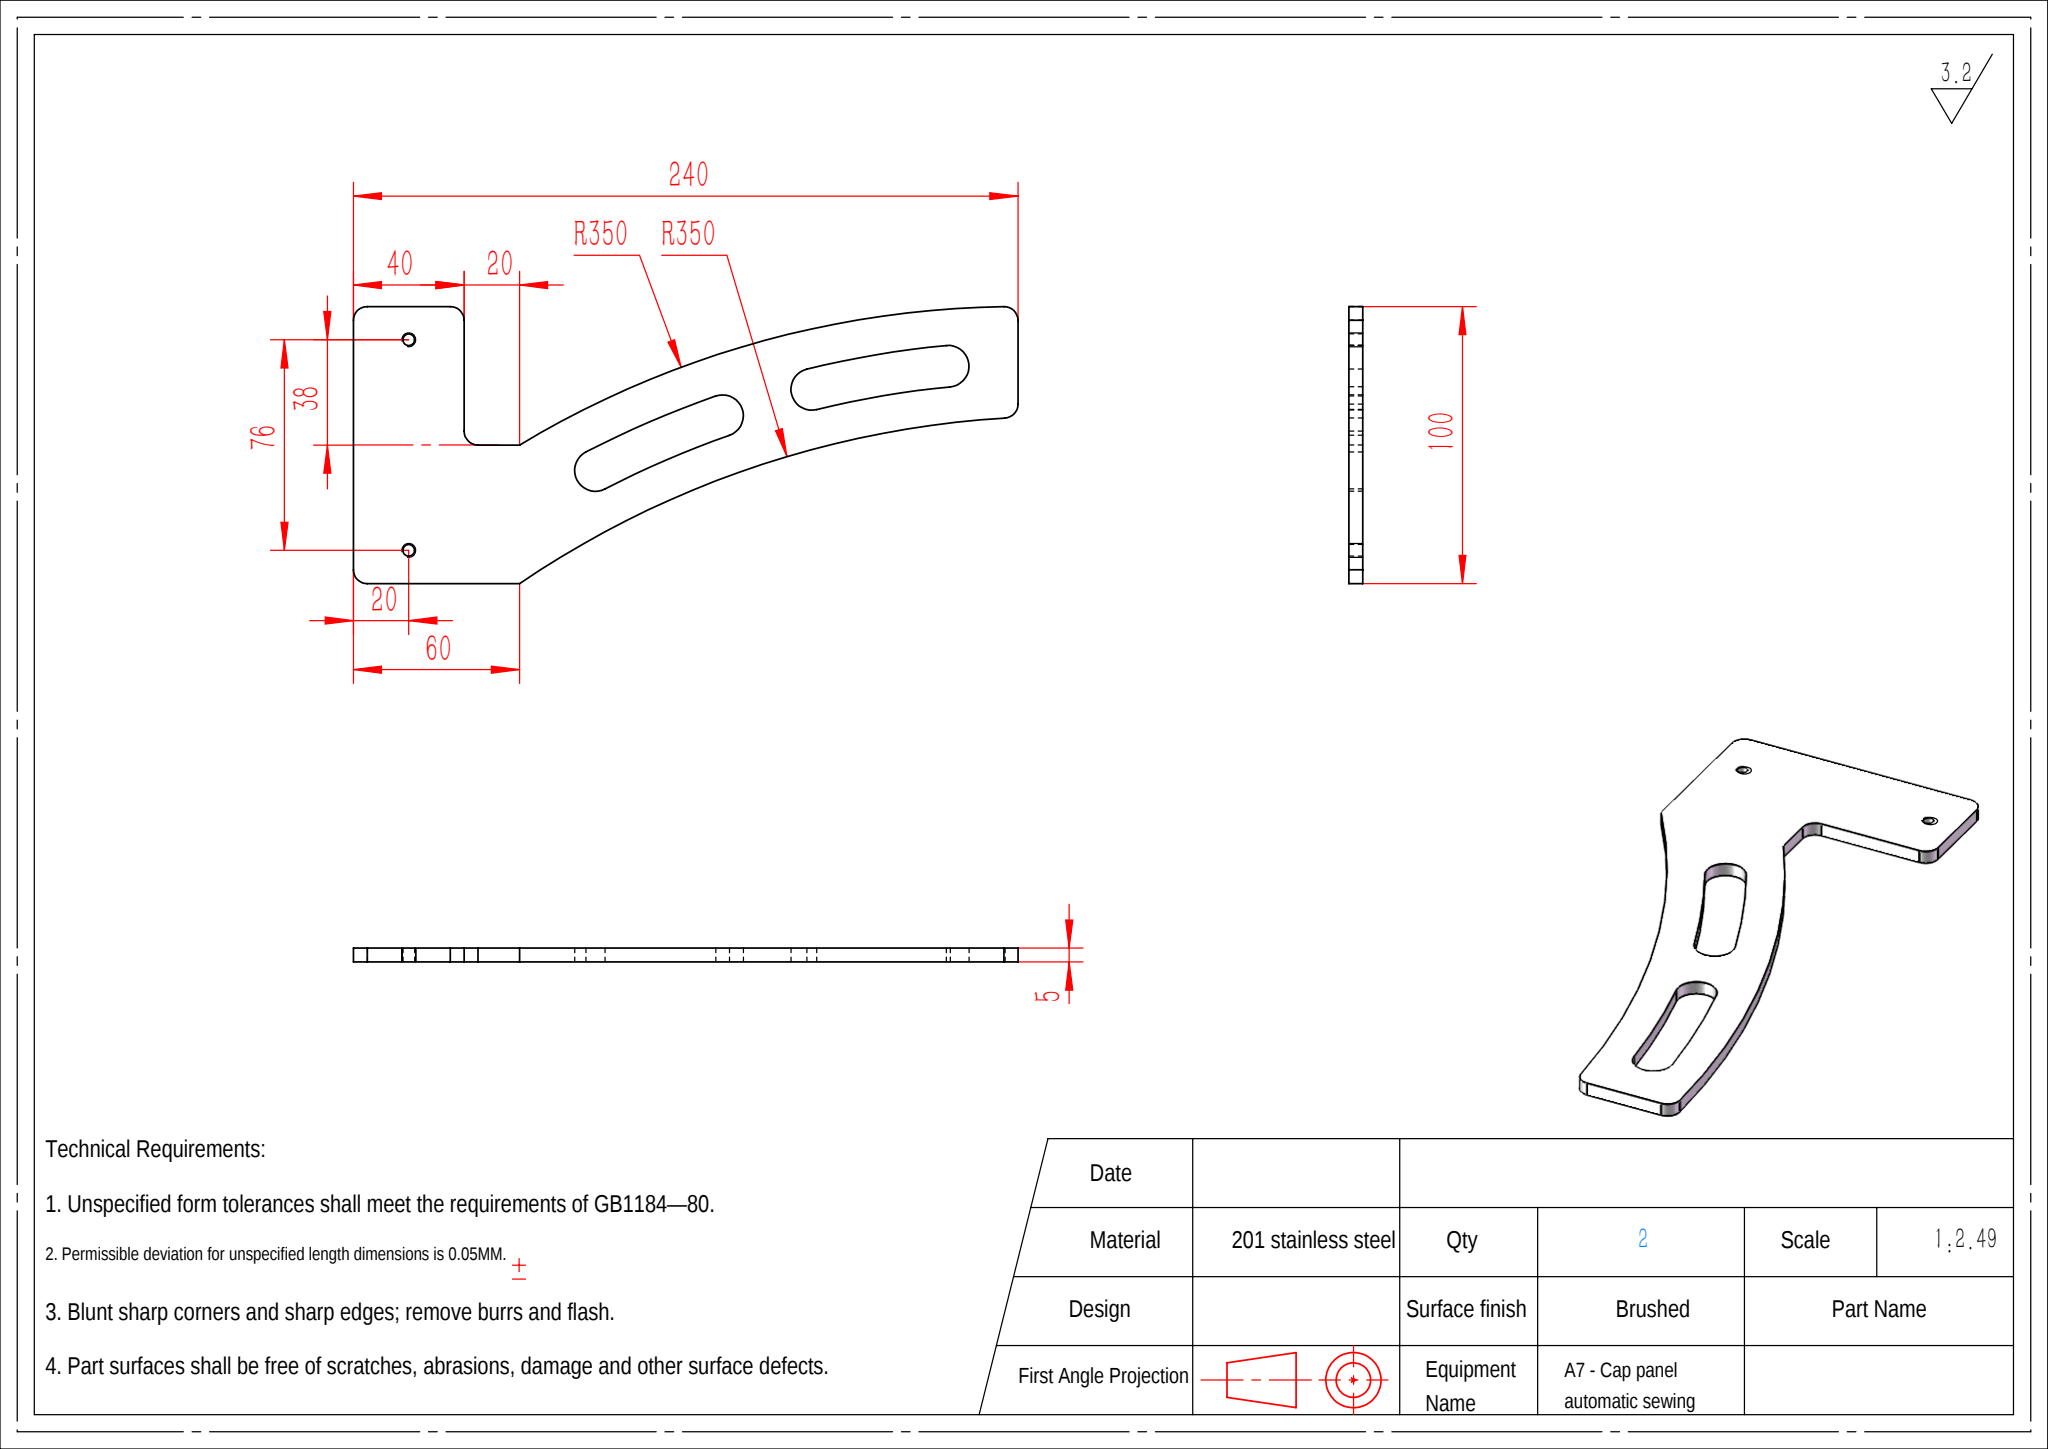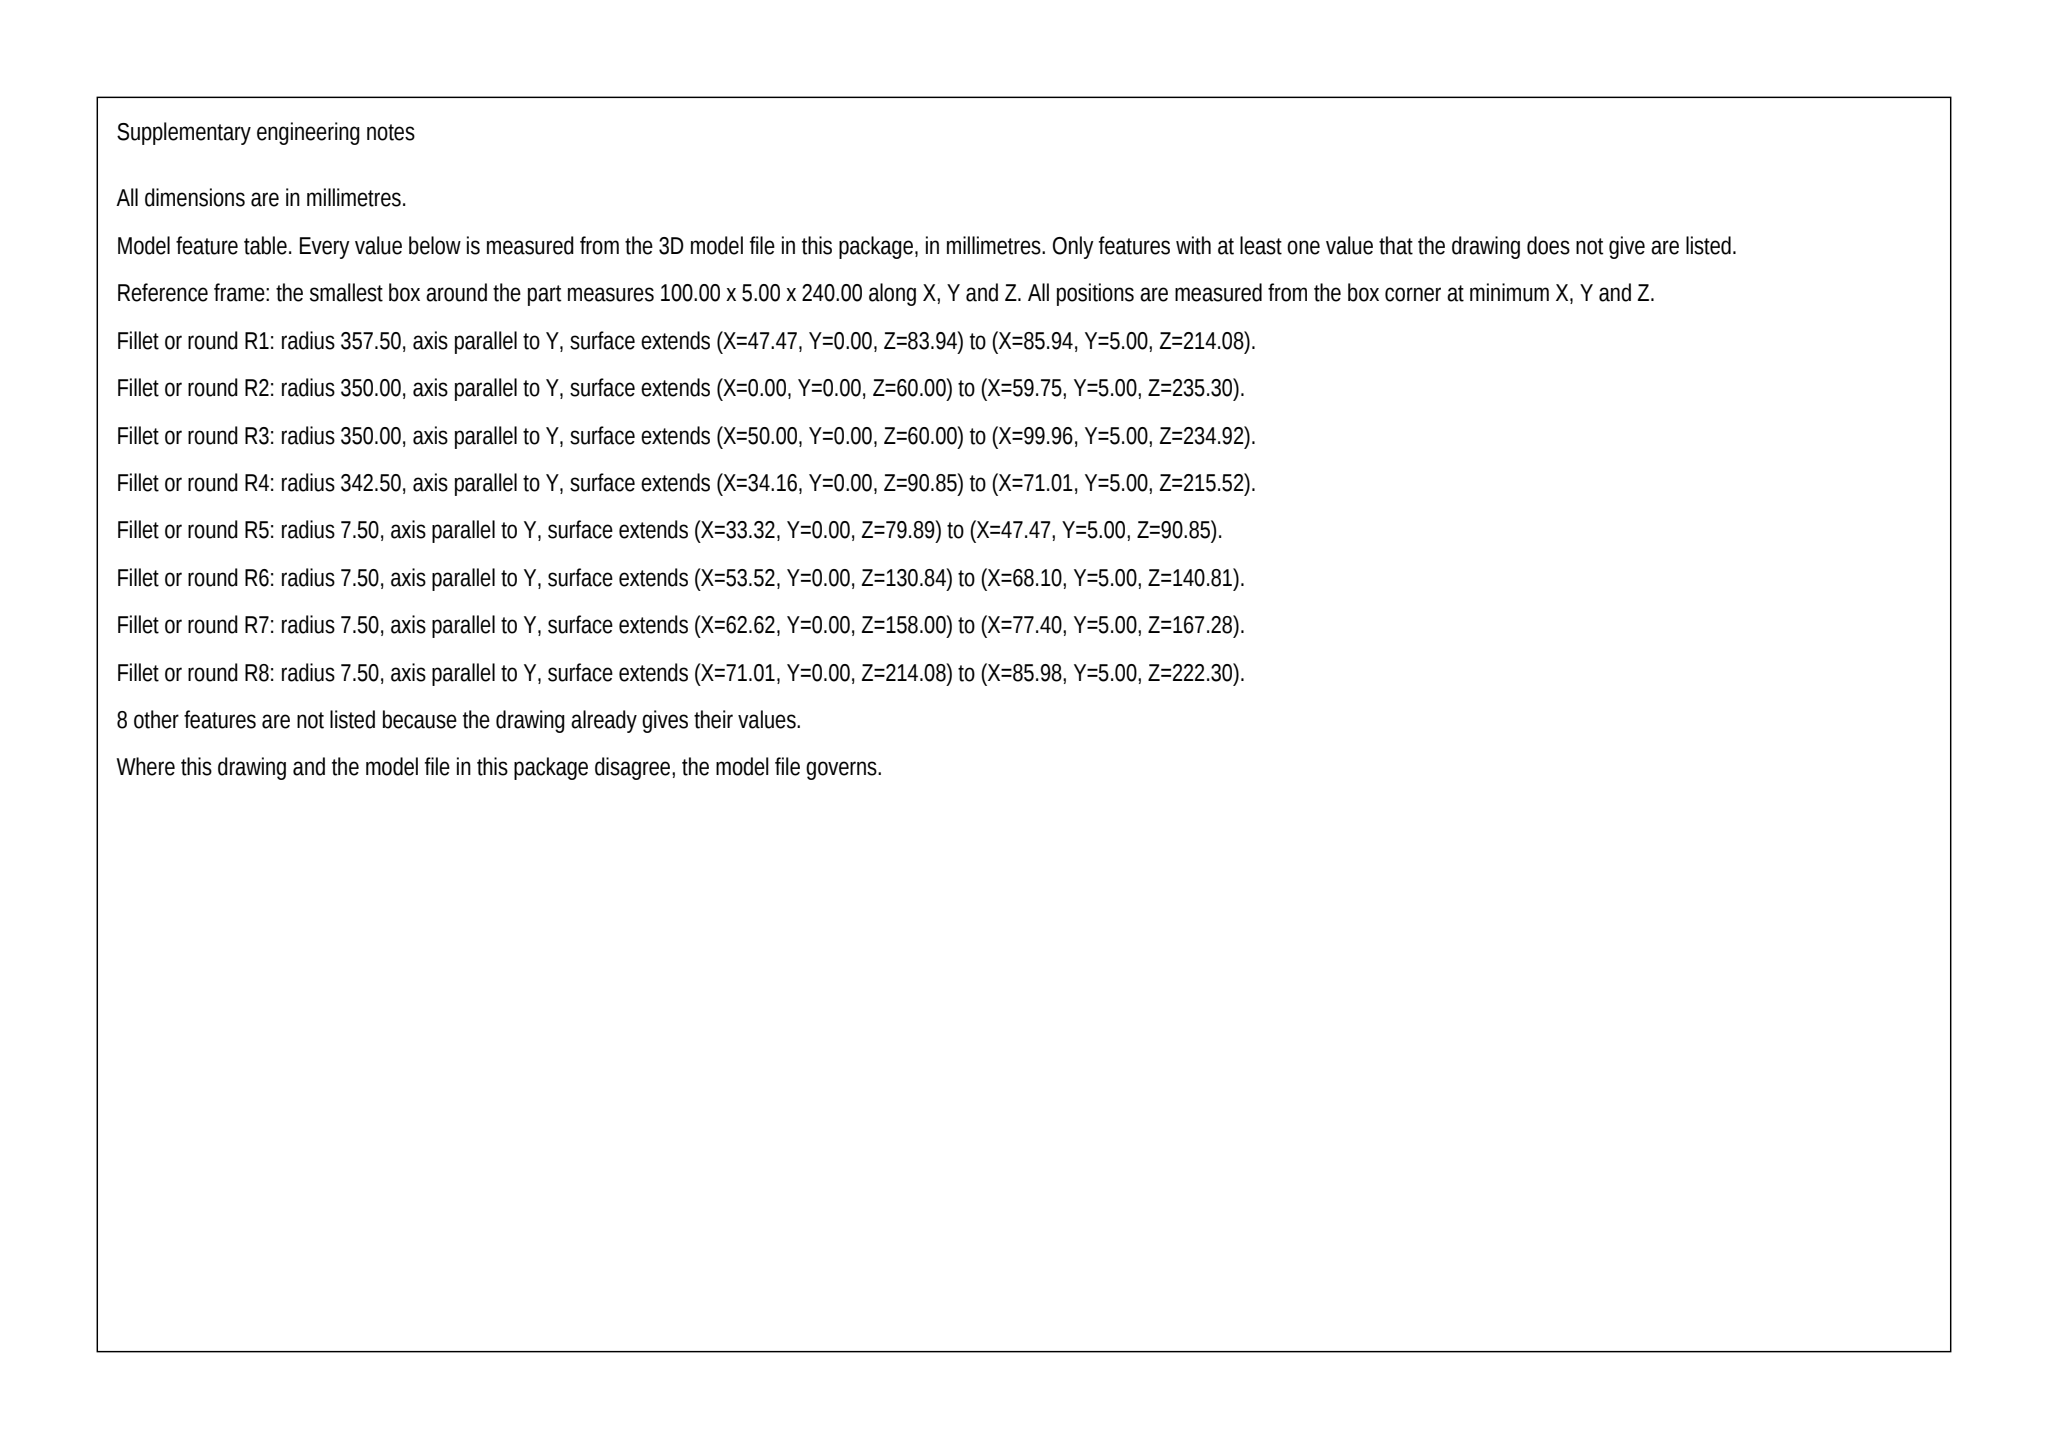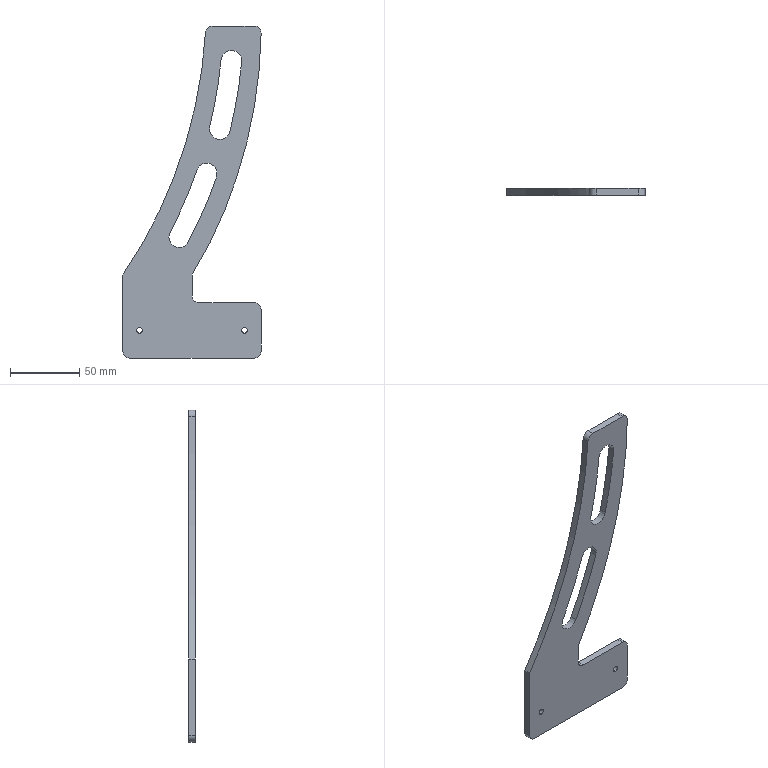Part | SolidWorks | mm | material 201 stainless steel | 1 solid | 30 faces | box 100 x 5 x 240 mm | volume 55599 mm3 | cylinder 22 | plane 8 | commonest cylinder face diameters 15 x6 10 x6 4.2 x4 700 x2 685 x2 715 x2
build123d program:
from build123d import *

# Parameters (mm, degrees)
SKETCH1_W           = 100
SKETCH1_H           = 240
BOSS_EXTRUDE1_DEPTH = 5
M5_TAPPED_HOLE1_D   = 4.2
CUT_EXTRUDE1_DEPTH  = 246.204
CUT_EXTRUDE2_DEPTH  = 246.204
SKETCH14_W          = 50
SKETCH14_H          = 20
CUT_EXTRUDE3_DEPTH  = 246.204
CUT_EXTRUDE4_DEPTH  = 246.204
FILLET1_R           = 5


with BuildPart() as part:
    # Sketch1 → Boss-Extrude1 (new body)
    with BuildSketch(Plane(origin=(0, 0, 0), x_dir=(1, 0, 0), z_dir=(0, 1, 0))):
        with Locations((0, -120)):
            Rectangle(SKETCH1_W, SKETCH1_H)
    extrude(amount=BOSS_EXTRUDE1_DEPTH)

    # M5 Tapped Hole1 (through all)
    with Locations(Plane(origin=(-38, 5, 20), x_dir=(0, 0, 1), z_dir=(0, 1, 0))):
        with Locations((0, 0)):
            m5_tapped_hole1 = Hole(M5_TAPPED_HOLE1_D / 2)

    # Mirror1: M5 Tapped Hole1 across plane
    add(m5_tapped_hole1.mirror(Plane(origin=(0, 0, 0), x_dir=(0, 0, 1), z_dir=(1, 0, 0))), mode=Mode.SUBTRACT)

    # Sketch7 → Cut-Extrude1 (cut, through all)
    with BuildSketch(Plane(origin=(0, 5, 0), x_dir=(1, 0, 0), z_dir=(0, 1, 0))):
        with BuildLine():
            Line((0, -60), (50, -60))
            Line((50, -60), (50, -240))
            ThreePointArc((50, -240), (37.231, -146.602), (0, -60))
        make_face()
    extrude(amount=-CUT_EXTRUDE1_DEPTH, mode=Mode.SUBTRACT)

    # Sketch11 → Cut-Extrude2 (cut, through all)
    with BuildSketch(Plane(origin=(0, 5, 0), x_dir=(1, 0, 0), z_dir=(0, 1, 0))):
        with BuildLine():
            Line((-50, -60), (-50, -240))
            Line((-50, -240), (10, -240))
            ThreePointArc((10, -240), (-7.57, -145.857), (-50, -60))
        make_face()
    extrude(amount=-CUT_EXTRUDE2_DEPTH, mode=Mode.SUBTRACT)

    # Sketch14 → Cut-Extrude3 (cut, through all)
    with BuildSketch(Plane(origin=(0, 5, 0), x_dir=(1, 0, 0), z_dir=(0, 1, 0))):
        with Locations((25, -50)):
            Rectangle(SKETCH14_W, SKETCH14_H)
    extrude(amount=-CUT_EXTRUDE3_DEPTH, mode=Mode.SUBTRACT)

    # Sketch15 → Cut-Extrude4 (cut, through all)
    with BuildSketch(Plane(origin=(0, 5, 0), x_dir=(1, 0, 0), z_dir=(0, 1, 0))):
        with BuildLine():
            ThreePointArc((17.685, -130.844), (8.418, -107.032), (-2.527, -83.942))
            ThreePointArc((-2.527, -83.942), (-12.637, -80.737), (-15.843, -90.847))
            ThreePointArc((-15.843, -90.847), (-5.358, -112.968), (3.52, -135.781))
            ThreePointArc((3.52, -135.781), (13.071, -140.395), (17.685, -130.844))
        make_face()
        with BuildLine():
            ThreePointArc((35.941, -214.075), (32.573, -188.746), (27.404, -163.722))
            ThreePointArc((27.404, -163.722), (18.339, -158.215), (12.831, -167.28))
            ThreePointArc((12.831, -167.28), (17.784, -191.254), (21.011, -215.52))
            ThreePointArc((21.011, -215.52), (29.198, -222.263), (35.941, -214.075))
        make_face()
    extrude(amount=-CUT_EXTRUDE4_DEPTH, mode=Mode.SUBTRACT)

    # Fillet1
    fillet1_edges = [part.edges().sort_by_distance(p)[0] for p in [
        (10, 2.5, 240),
        (0, 2.5, 40),
        (50, 2.5, 40),
        (-50, 2.5, 0),
        (50, 2.5, 0),
        (50, 2.5, 240),
    ]]
    fillet(fillet1_edges, radius=FILLET1_R)


solid = part.part